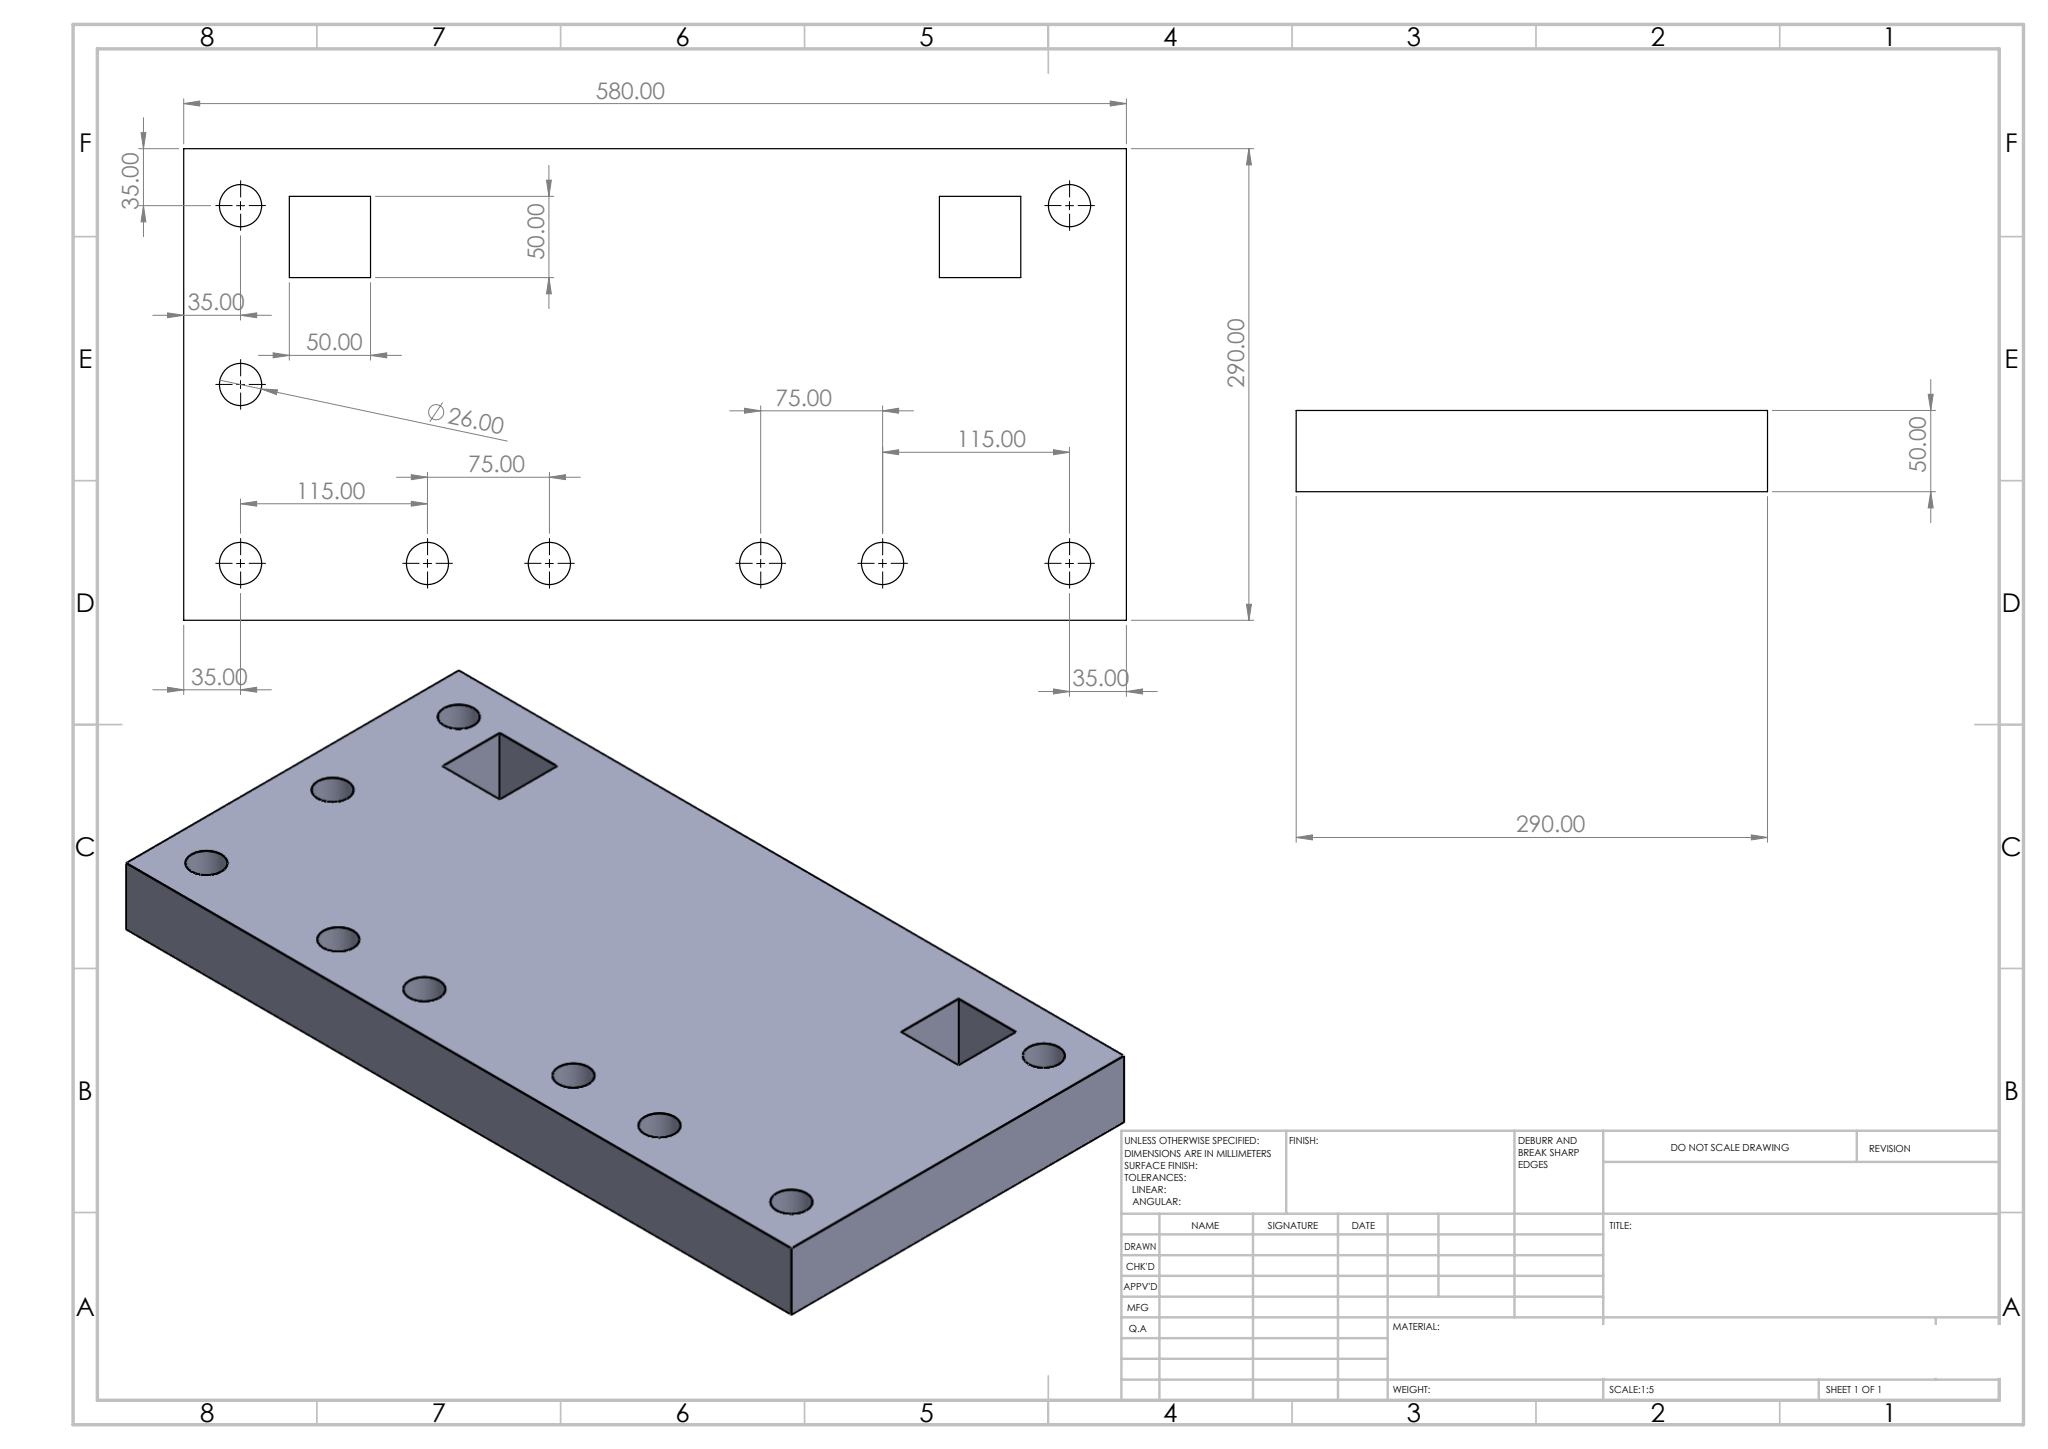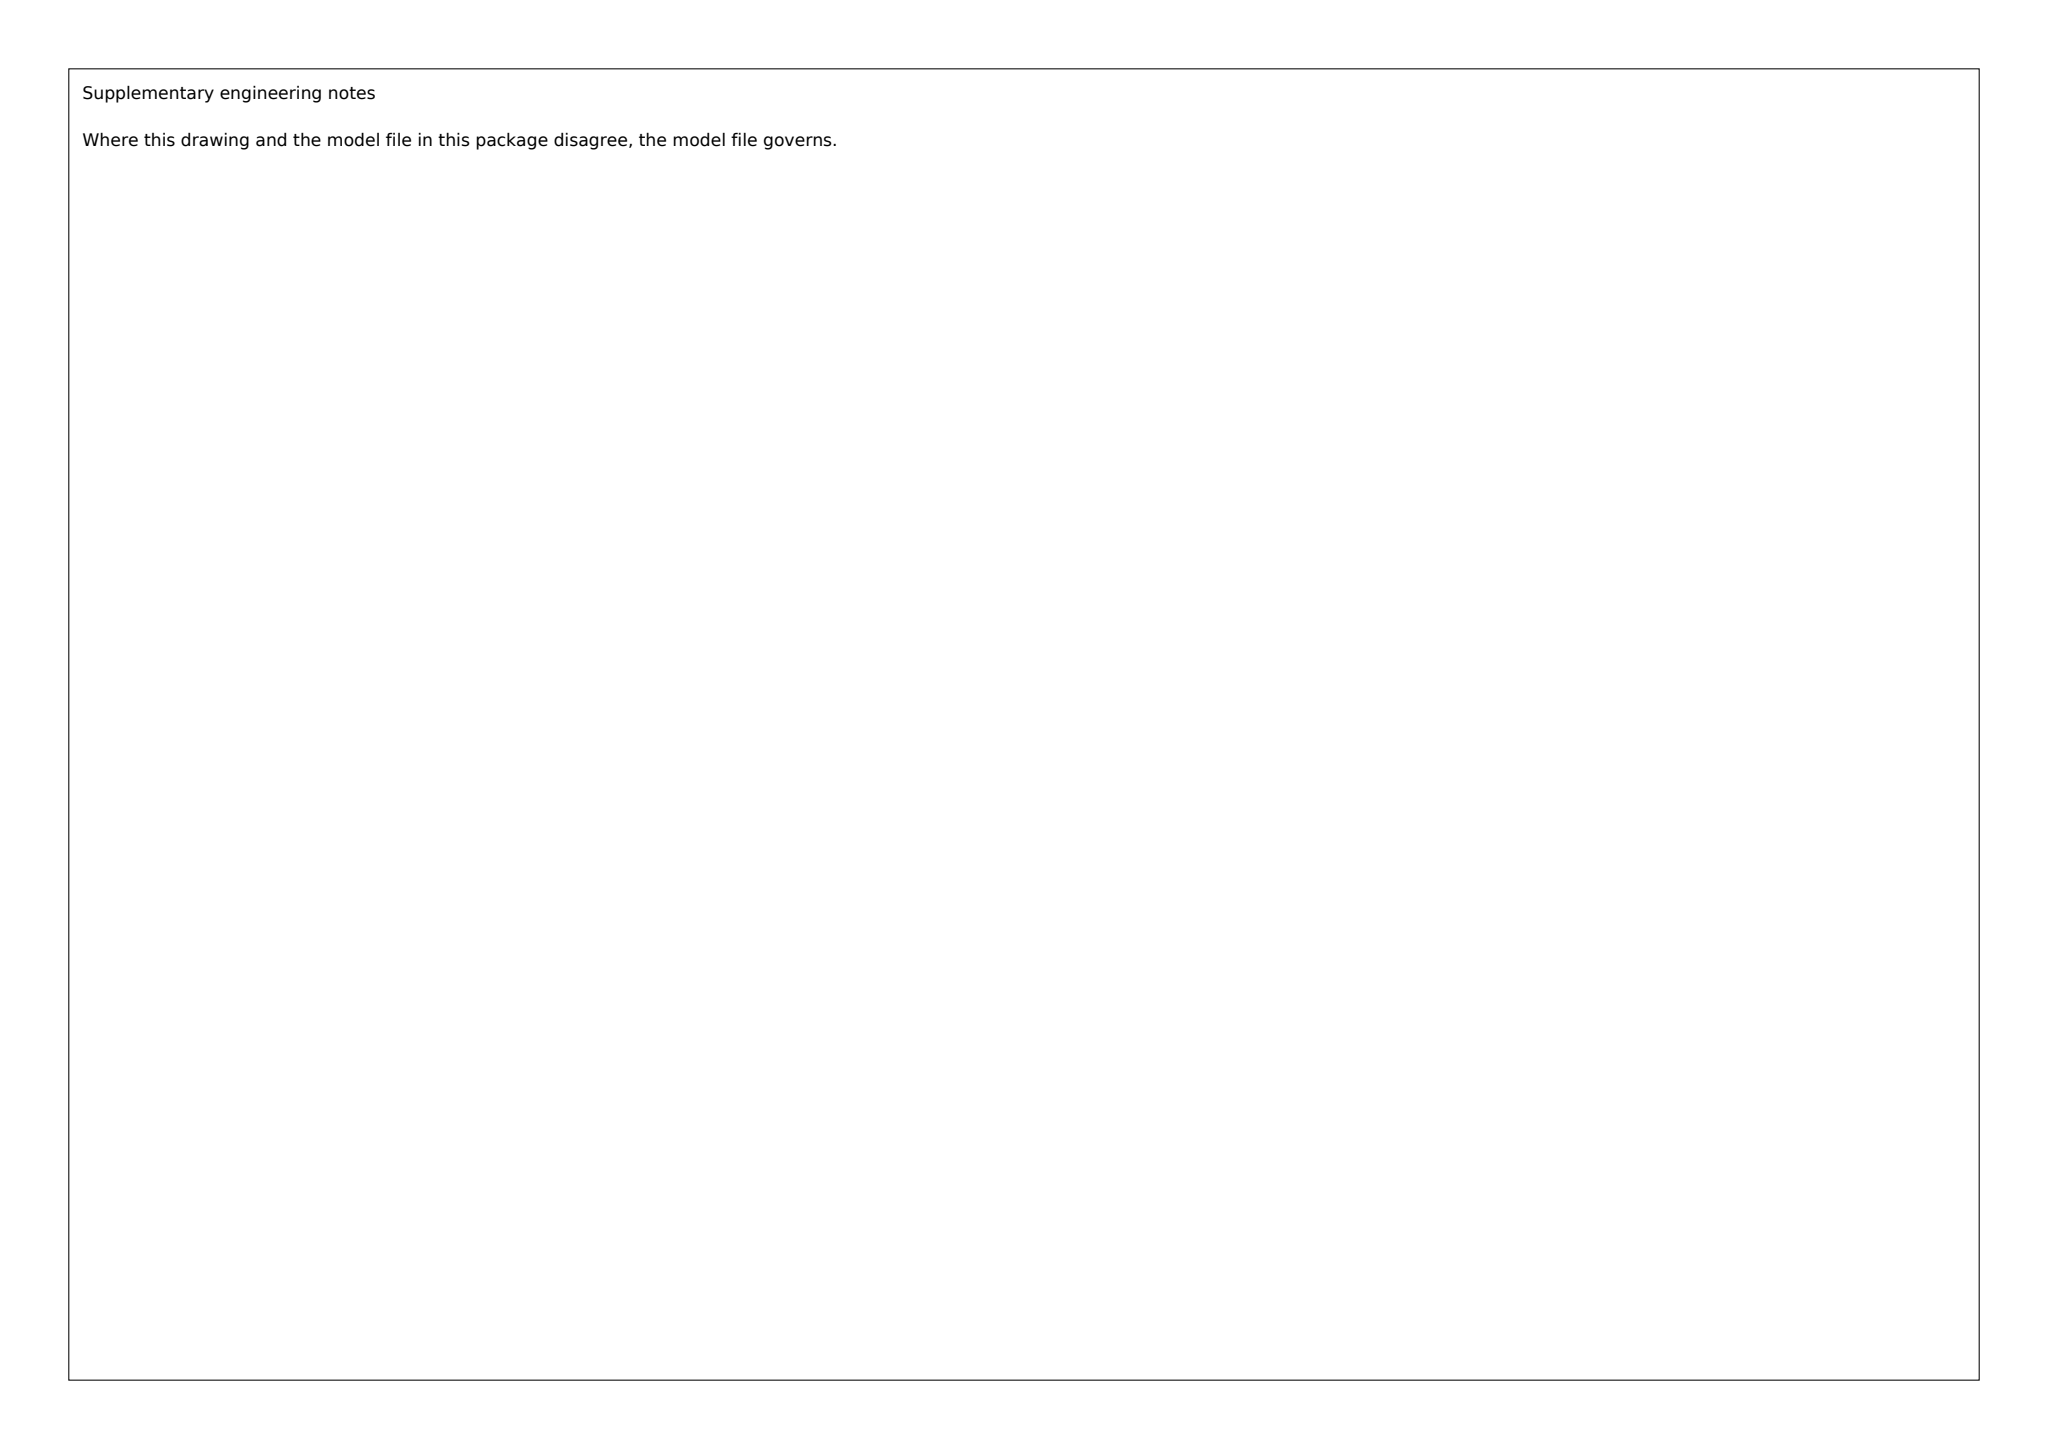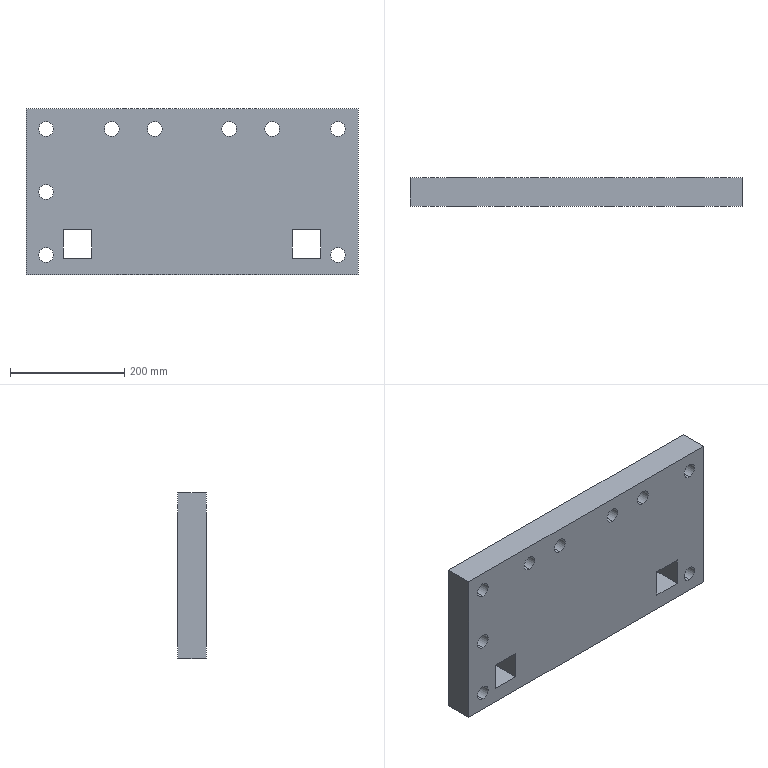Part | SolidWorks | mm | 1 solid | 32 faces | box 580 x 50 x 290 mm | volume 7921082 mm3 | cylinder 18 | plane 14 | commonest cylinder face diameters 26 x18
Drawing notes:
FRONT VIEW: BOTTOM ROW 6X Ø26 HOLES 35 FROM BOTTOM EDGE | from the solid: Ø26 cyl axes at z=255 with bbox z=290 → 290-255=35 from bottom edge
build123d program:
from build123d import *

# Parameters (mm, degrees)
SKETCH2_W           = 580
SKETCH2_H           = 290
SKETCH2_R           = 13
BOSS_EXTRUDE1_DEPTH = 50
SKETCH3_W           = 50
SKETCH3_H           = 50
CUT_EXTRUDE1_DEPTH  = 329.062


with BuildPart() as part:
    # Sketch2 → Boss-Extrude1 (new body)
    with BuildSketch(Plane(origin=(0, 0, 0), x_dir=(1, 0, 0), z_dir=(0, 1, 0))):
        Rectangle(SKETCH2_W, SKETCH2_H)
        with Locations(Location((-255, -110, 0), (0, 0, 270))):
            Circle(SKETCH2_R, mode=Mode.SUBTRACT)
        with Locations(Location((-140, -110, 0), (0, 0, 270))):
            Circle(SKETCH2_R, mode=Mode.SUBTRACT)
        with Locations(Location((-65, -110, 0), (0, 0, 270))):
            Circle(SKETCH2_R, mode=Mode.SUBTRACT)
        with Locations(Location((65, -110, 0), (0, 0, 270))):
            Circle(SKETCH2_R, mode=Mode.SUBTRACT)
        with Locations(Location((140, -110, 0), (0, 0, 270))):
            Circle(SKETCH2_R, mode=Mode.SUBTRACT)
        with Locations(Location((255, -110, 0), (0, 0, 270))):
            Circle(SKETCH2_R, mode=Mode.SUBTRACT)
        with Locations(Location((-255, 0, 0), (0, 0, 270))):
            Circle(SKETCH2_R, mode=Mode.SUBTRACT)
        with Locations(Location((-255, 110, 0), (0, 0, 270))):
            Circle(SKETCH2_R, mode=Mode.SUBTRACT)
        with Locations(Location((255, 110, 0), (0, 0, 270))):
            Circle(SKETCH2_R, mode=Mode.SUBTRACT)
    extrude(amount=BOSS_EXTRUDE1_DEPTH)

    # Sketch3 → Cut-Extrude1 (cut, through all)
    with BuildSketch(Plane(origin=(0, 50, 0), x_dir=(1, 0, 0), z_dir=(0, 1, 0))):
        with Locations((200, 90.71)):
            Rectangle(SKETCH3_W, SKETCH3_H)
        with Locations((-200, 90.71)):
            Rectangle(SKETCH3_W, SKETCH3_H)
    extrude(amount=-CUT_EXTRUDE1_DEPTH, mode=Mode.SUBTRACT)


solid = part.part